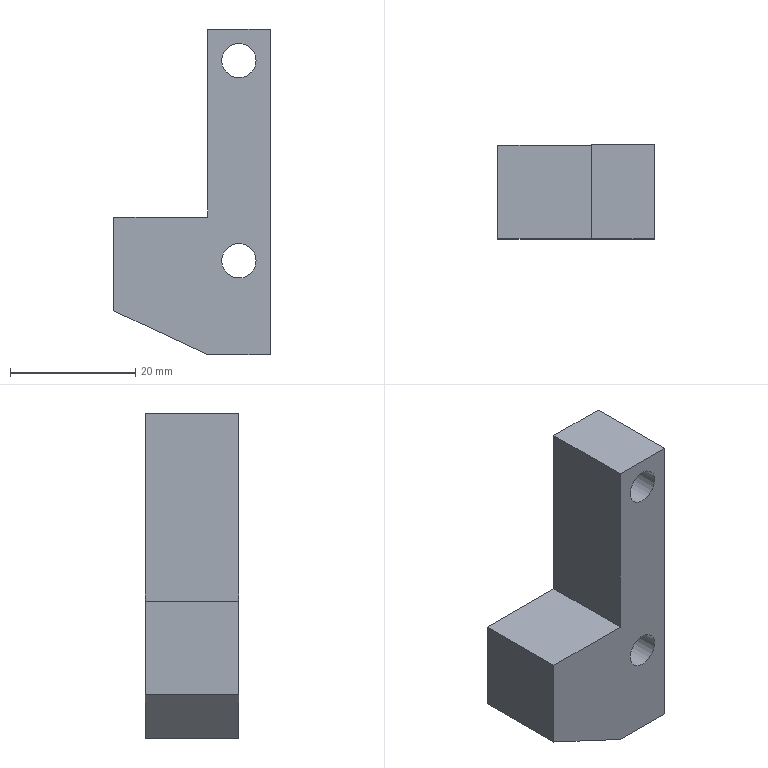Component | NX | NYLON_STOPPER_BLOCK_2 | 1 solid | 11 faces | box 25 x 15 x 52 mm | volume 11250 mm3 | plane 9 | cylinder 2 | commonest cylinder face diameters 5.5 x2
STEP:
#1=CARTESIAN_POINT('',(0.,0.,0.));
#2=DIRECTION('',(0.,0.,1.));
#3=DIRECTION('',(1.,0.,0.));
#4=AXIS2_PLACEMENT_3D('',#1,#2,#3);
#5=CARTESIAN_POINT('',(127.866,114.757,126.466));
#6=VERTEX_POINT('',#5);
#7=CARTESIAN_POINT('',(127.866,114.757,74.466));
#8=VERTEX_POINT('',#7);
#9=CARTESIAN_POINT('',(127.866,114.757,126.466));
#10=DIRECTION('',(0.,0.,-1.));
#11=VECTOR('',#10,1.);
#12=LINE('',#9,#11);
#13=CARTESIAN_POINT('',(127.866,129.757,126.466));
#14=DIRECTION('',(-1.,0.,0.));
#15=DIRECTION('',(0.,-1.,0.));
#16=AXIS2_PLACEMENT_3D('',#13,#14,#15);
#17=PLANE('',#16);
#18=CARTESIAN_POINT('',(15.,0.));
#19=DIRECTION('',(0.,-1.));
#20=VECTOR('',#19,1.);
#21=LINE('',#18,#20);
#22=(GEOMETRIC_REPRESENTATION_CONTEXT(2)PARAMETRIC_REPRESENTATION_CONTEXT()REPRESENTATION_CONTEXT('',''));
#23=DEFINITIONAL_REPRESENTATION('',(#21),#22);
#24=PCURVE('',#17,#23);
#25=CARTESIAN_POINT('',(122.866,114.757,89.466));
#26=DIRECTION('',(0.,1.,0.));
#27=DIRECTION('',(-1.,0.,0.));
#28=AXIS2_PLACEMENT_3D('',#25,#26,#27);
#29=PLANE('',#28);
#30=CARTESIAN_POINT('',(-5.,37.));
#31=DIRECTION('',(0.,-1.));
#32=VECTOR('',#31,1.);
#33=LINE('',#30,#32);
#34=(GEOMETRIC_REPRESENTATION_CONTEXT(2)PARAMETRIC_REPRESENTATION_CONTEXT()REPRESENTATION_CONTEXT('',''));
#35=DEFINITIONAL_REPRESENTATION('',(#33),#34);
#36=PCURVE('',#29,#35);
#37=SURFACE_CURVE('',#12,(#24,#36),.PCURVE_S1.);
#38=EDGE_CURVE('',#6,#8,#37,.T.);
#39=ORIENTED_EDGE('',*,*,#38,.T.);
#40=CARTESIAN_POINT('',(127.866,129.757,74.466));
#41=VERTEX_POINT('',#40);
#42=CARTESIAN_POINT('',(127.866,129.757,74.466));
#43=DIRECTION('',(0.,-1.,0.));
#44=VECTOR('',#43,1.);
#45=LINE('',#42,#44);
#46=CARTESIAN_POINT('',(0.,-52.));
#47=DIRECTION('',(1.,0.));
#48=VECTOR('',#47,1.);
#49=LINE('',#46,#48);
#50=(GEOMETRIC_REPRESENTATION_CONTEXT(2)PARAMETRIC_REPRESENTATION_CONTEXT()REPRESENTATION_CONTEXT('',''));
#51=DEFINITIONAL_REPRESENTATION('',(#49),#50);
#52=PCURVE('',#17,#51);
#53=CARTESIAN_POINT('',(127.866,129.757,74.466));
#54=DIRECTION('',(0.,0.,1.));
#55=DIRECTION('',(0.,1.,0.));
#56=AXIS2_PLACEMENT_3D('',#53,#54,#55);
#57=PLANE('',#56);
#58=CARTESIAN_POINT('',(0.,0.));
#59=DIRECTION('',(-1.,0.));
#60=VECTOR('',#59,1.);
#61=LINE('',#58,#60);
#62=(GEOMETRIC_REPRESENTATION_CONTEXT(2)PARAMETRIC_REPRESENTATION_CONTEXT()REPRESENTATION_CONTEXT('',''));
#63=DEFINITIONAL_REPRESENTATION('',(#61),#62);
#64=PCURVE('',#57,#63);
#65=SURFACE_CURVE('',#45,(#52,#64),.PCURVE_S1.);
#66=EDGE_CURVE('',#41,#8,#65,.T.);
#67=ORIENTED_EDGE('',*,*,#66,.F.);
#68=CARTESIAN_POINT('',(127.866,129.757,126.466));
#69=VERTEX_POINT('',#68);
#70=CARTESIAN_POINT('',(127.866,129.757,126.466));
#71=DIRECTION('',(0.,0.,-1.));
#72=VECTOR('',#71,1.);
#73=LINE('',#70,#72);
#74=CARTESIAN_POINT('',(0.,0.));
#75=DIRECTION('',(0.,-1.));
#76=VECTOR('',#75,1.);
#77=LINE('',#74,#76);
#78=(GEOMETRIC_REPRESENTATION_CONTEXT(2)PARAMETRIC_REPRESENTATION_CONTEXT()REPRESENTATION_CONTEXT('',''));
#79=DEFINITIONAL_REPRESENTATION('',(#77),#78);
#80=PCURVE('',#17,#79);
#81=CARTESIAN_POINT('',(122.866,129.757,89.466));
#82=DIRECTION('',(0.,1.,0.));
#83=DIRECTION('',(-1.,0.,0.));
#84=AXIS2_PLACEMENT_3D('',#81,#82,#83);
#85=PLANE('',#84);
#86=CARTESIAN_POINT('',(-5.,37.));
#87=DIRECTION('',(0.,-1.));
#88=VECTOR('',#87,1.);
#89=LINE('',#86,#88);
#90=(GEOMETRIC_REPRESENTATION_CONTEXT(2)PARAMETRIC_REPRESENTATION_CONTEXT()REPRESENTATION_CONTEXT('',''));
#91=DEFINITIONAL_REPRESENTATION('',(#89),#90);
#92=PCURVE('',#85,#91);
#93=SURFACE_CURVE('',#73,(#80,#92),.PCURVE_S1.);
#94=EDGE_CURVE('',#69,#41,#93,.T.);
#95=ORIENTED_EDGE('',*,*,#94,.F.);
#96=CARTESIAN_POINT('',(127.866,129.757,126.466));
#97=DIRECTION('',(0.,-1.,0.));
#98=VECTOR('',#97,1.);
#99=LINE('',#96,#98);
#100=CARTESIAN_POINT('',(0.,0.));
#101=DIRECTION('',(1.,0.));
#102=VECTOR('',#101,1.);
#103=LINE('',#100,#102);
#104=(GEOMETRIC_REPRESENTATION_CONTEXT(2)PARAMETRIC_REPRESENTATION_CONTEXT()REPRESENTATION_CONTEXT('',''));
#105=DEFINITIONAL_REPRESENTATION('',(#103),#104);
#106=PCURVE('',#17,#105);
#107=CARTESIAN_POINT('',(117.866,129.757,126.466));
#108=DIRECTION('',(0.,0.,-1.));
#109=DIRECTION('',(0.,-1.,0.));
#110=AXIS2_PLACEMENT_3D('',#107,#108,#109);
#111=PLANE('',#110);
#112=CARTESIAN_POINT('',(0.,-10.));
#113=DIRECTION('',(1.,0.));
#114=VECTOR('',#113,1.);
#115=LINE('',#112,#114);
#116=(GEOMETRIC_REPRESENTATION_CONTEXT(2)PARAMETRIC_REPRESENTATION_CONTEXT()REPRESENTATION_CONTEXT('',''));
#117=DEFINITIONAL_REPRESENTATION('',(#115),#116);
#118=PCURVE('',#111,#117);
#119=SURFACE_CURVE('',#99,(#106,#118),.PCURVE_S1.);
#120=EDGE_CURVE('',#69,#6,#119,.T.);
#121=ORIENTED_EDGE('',*,*,#120,.T.);
#122=EDGE_LOOP('',(#39,#67,#95,#121));
#123=FACE_BOUND('',#122,.T.);
#124=ADVANCED_FACE('',(#123),#17,.F.);
#125=CARTESIAN_POINT('',(117.866,114.757,74.466));
#126=VERTEX_POINT('',#125);
#127=CARTESIAN_POINT('',(127.866,114.757,74.466));
#128=DIRECTION('',(-1.,0.,0.));
#129=VECTOR('',#128,1.);
#130=LINE('',#127,#129);
#131=CARTESIAN_POINT('',(-15.,0.));
#132=DIRECTION('',(0.,1.));
#133=VECTOR('',#132,1.);
#134=LINE('',#131,#133);
#135=(GEOMETRIC_REPRESENTATION_CONTEXT(2)PARAMETRIC_REPRESENTATION_CONTEXT()REPRESENTATION_CONTEXT('',''));
#136=DEFINITIONAL_REPRESENTATION('',(#134),#135);
#137=PCURVE('',#57,#136);
#138=CARTESIAN_POINT('',(-5.,-15.));
#139=DIRECTION('',(1.,0.));
#140=VECTOR('',#139,1.);
#141=LINE('',#138,#140);
#142=(GEOMETRIC_REPRESENTATION_CONTEXT(2)PARAMETRIC_REPRESENTATION_CONTEXT()REPRESENTATION_CONTEXT('',''));
#143=DEFINITIONAL_REPRESENTATION('',(#141),#142);
#144=PCURVE('',#29,#143);
#145=SURFACE_CURVE('',#130,(#137,#144),.PCURVE_S1.);
#146=EDGE_CURVE('',#8,#126,#145,.T.);
#147=ORIENTED_EDGE('',*,*,#146,.T.);
#148=CARTESIAN_POINT('',(117.866,129.757,74.466));
#149=VERTEX_POINT('',#148);
#150=CARTESIAN_POINT('',(117.866,129.757,74.466));
#151=DIRECTION('',(0.,-1.,0.));
#152=VECTOR('',#151,1.);
#153=LINE('',#150,#152);
#154=CARTESIAN_POINT('',(0.,10.));
#155=DIRECTION('',(-1.,0.));
#156=VECTOR('',#155,1.);
#157=LINE('',#154,#156);
#158=(GEOMETRIC_REPRESENTATION_CONTEXT(2)PARAMETRIC_REPRESENTATION_CONTEXT()REPRESENTATION_CONTEXT('',''));
#159=DEFINITIONAL_REPRESENTATION('',(#157),#158);
#160=PCURVE('',#57,#159);
#161=CARTESIAN_POINT('',(117.866,129.757,74.466));
#162=DIRECTION('',(0.4229,0.,0.9062));
#163=DIRECTION('',(0.9062,0.,-0.4229));
#164=AXIS2_PLACEMENT_3D('',#161,#162,#163);
#165=PLANE('',#164);
#166=CARTESIAN_POINT('',(0.,0.));
#167=DIRECTION('',(0.,-1.));
#168=VECTOR('',#167,1.);
#169=LINE('',#166,#168);
#170=(GEOMETRIC_REPRESENTATION_CONTEXT(2)PARAMETRIC_REPRESENTATION_CONTEXT()REPRESENTATION_CONTEXT('',''));
#171=DEFINITIONAL_REPRESENTATION('',(#169),#170);
#172=PCURVE('',#165,#171);
#173=SURFACE_CURVE('',#153,(#160,#172),.PCURVE_S1.);
#174=EDGE_CURVE('',#149,#126,#173,.T.);
#175=ORIENTED_EDGE('',*,*,#174,.F.);
#176=CARTESIAN_POINT('',(127.866,129.757,74.466));
#177=DIRECTION('',(-1.,0.,0.));
#178=VECTOR('',#177,1.);
#179=LINE('',#176,#178);
#180=CARTESIAN_POINT('',(0.,0.));
#181=DIRECTION('',(0.,1.));
#182=VECTOR('',#181,1.);
#183=LINE('',#180,#182);
#184=(GEOMETRIC_REPRESENTATION_CONTEXT(2)PARAMETRIC_REPRESENTATION_CONTEXT()REPRESENTATION_CONTEXT('',''));
#185=DEFINITIONAL_REPRESENTATION('',(#183),#184);
#186=PCURVE('',#57,#185);
#187=CARTESIAN_POINT('',(-5.,-15.));
#188=DIRECTION('',(1.,0.));
#189=VECTOR('',#188,1.);
#190=LINE('',#187,#189);
#191=(GEOMETRIC_REPRESENTATION_CONTEXT(2)PARAMETRIC_REPRESENTATION_CONTEXT()REPRESENTATION_CONTEXT('',''));
#192=DEFINITIONAL_REPRESENTATION('',(#190),#191);
#193=PCURVE('',#85,#192);
#194=SURFACE_CURVE('',#179,(#186,#193),.PCURVE_S1.);
#195=EDGE_CURVE('',#41,#149,#194,.T.);
#196=ORIENTED_EDGE('',*,*,#195,.F.);
#197=ORIENTED_EDGE('',*,*,#66,.T.);
#198=EDGE_LOOP('',(#147,#175,#196,#197));
#199=FACE_BOUND('',#198,.T.);
#200=ADVANCED_FACE('',(#199),#57,.F.);
#201=CARTESIAN_POINT('',(102.866,114.757,81.466));
#202=VERTEX_POINT('',#201);
#203=CARTESIAN_POINT('',(117.866,114.757,74.466));
#204=DIRECTION('',(-0.9062,0.,0.4229));
#205=VECTOR('',#204,1.);
#206=LINE('',#203,#205);
#207=CARTESIAN_POINT('',(0.,-15.));
#208=DIRECTION('',(-1.,0.));
#209=VECTOR('',#208,1.);
#210=LINE('',#207,#209);
#211=(GEOMETRIC_REPRESENTATION_CONTEXT(2)PARAMETRIC_REPRESENTATION_CONTEXT()REPRESENTATION_CONTEXT('',''));
#212=DEFINITIONAL_REPRESENTATION('',(#210),#211);
#213=PCURVE('',#165,#212);
#214=CARTESIAN_POINT('',(5.,-15.));
#215=DIRECTION('',(0.9062,0.4229));
#216=VECTOR('',#215,1.);
#217=LINE('',#214,#216);
#218=(GEOMETRIC_REPRESENTATION_CONTEXT(2)PARAMETRIC_REPRESENTATION_CONTEXT()REPRESENTATION_CONTEXT('',''));
#219=DEFINITIONAL_REPRESENTATION('',(#217),#218);
#220=PCURVE('',#29,#219);
#221=SURFACE_CURVE('',#206,(#213,#220),.PCURVE_S1.);
#222=EDGE_CURVE('',#126,#202,#221,.T.);
#223=ORIENTED_EDGE('',*,*,#222,.T.);
#224=CARTESIAN_POINT('',(102.866,129.757,81.466));
#225=VERTEX_POINT('',#224);
#226=CARTESIAN_POINT('',(102.866,129.757,81.466));
#227=DIRECTION('',(0.,-1.,0.));
#228=VECTOR('',#227,1.);
#229=LINE('',#226,#228);
#230=CARTESIAN_POINT('',(-16.553,0.));
#231=DIRECTION('',(0.,-1.));
#232=VECTOR('',#231,1.);
#233=LINE('',#230,#232);
#234=(GEOMETRIC_REPRESENTATION_CONTEXT(2)PARAMETRIC_REPRESENTATION_CONTEXT()REPRESENTATION_CONTEXT('',''));
#235=DEFINITIONAL_REPRESENTATION('',(#233),#234);
#236=PCURVE('',#165,#235);
#237=CARTESIAN_POINT('',(102.866,129.757,81.466));
#238=DIRECTION('',(1.,0.,-0.));
#239=DIRECTION('',(-0.,0.,-1.));
#240=AXIS2_PLACEMENT_3D('',#237,#238,#239);
#241=PLANE('',#240);
#242=CARTESIAN_POINT('',(0.,0.));
#243=DIRECTION('',(0.,-1.));
#244=VECTOR('',#243,1.);
#245=LINE('',#242,#244);
#246=(GEOMETRIC_REPRESENTATION_CONTEXT(2)PARAMETRIC_REPRESENTATION_CONTEXT()REPRESENTATION_CONTEXT('',''));
#247=DEFINITIONAL_REPRESENTATION('',(#245),#246);
#248=PCURVE('',#241,#247);
#249=SURFACE_CURVE('',#229,(#236,#248),.PCURVE_S1.);
#250=EDGE_CURVE('',#225,#202,#249,.T.);
#251=ORIENTED_EDGE('',*,*,#250,.F.);
#252=CARTESIAN_POINT('',(117.866,129.757,74.466));
#253=DIRECTION('',(-0.9062,0.,0.4229));
#254=VECTOR('',#253,1.);
#255=LINE('',#252,#254);
#256=CARTESIAN_POINT('',(0.,0.));
#257=DIRECTION('',(-1.,0.));
#258=VECTOR('',#257,1.);
#259=LINE('',#256,#258);
#260=(GEOMETRIC_REPRESENTATION_CONTEXT(2)PARAMETRIC_REPRESENTATION_CONTEXT()REPRESENTATION_CONTEXT('',''));
#261=DEFINITIONAL_REPRESENTATION('',(#259),#260);
#262=PCURVE('',#165,#261);
#263=CARTESIAN_POINT('',(5.,-15.));
#264=DIRECTION('',(0.9062,0.4229));
#265=VECTOR('',#264,1.);
#266=LINE('',#263,#265);
#267=(GEOMETRIC_REPRESENTATION_CONTEXT(2)PARAMETRIC_REPRESENTATION_CONTEXT()REPRESENTATION_CONTEXT('',''));
#268=DEFINITIONAL_REPRESENTATION('',(#266),#267);
#269=PCURVE('',#85,#268);
#270=SURFACE_CURVE('',#255,(#262,#269),.PCURVE_S1.);
#271=EDGE_CURVE('',#149,#225,#270,.T.);
#272=ORIENTED_EDGE('',*,*,#271,.F.);
#273=ORIENTED_EDGE('',*,*,#174,.T.);
#274=EDGE_LOOP('',(#223,#251,#272,#273));
#275=FACE_BOUND('',#274,.T.);
#276=ADVANCED_FACE('',(#275),#165,.F.);
#277=CARTESIAN_POINT('',(102.866,114.757,96.466));
#278=VERTEX_POINT('',#277);
#279=CARTESIAN_POINT('',(102.866,114.757,81.466));
#280=DIRECTION('',(0.,0.,1.));
#281=VECTOR('',#280,1.);
#282=LINE('',#279,#281);
#283=CARTESIAN_POINT('',(0.,-15.));
#284=DIRECTION('',(-1.,0.));
#285=VECTOR('',#284,1.);
#286=LINE('',#283,#285);
#287=(GEOMETRIC_REPRESENTATION_CONTEXT(2)PARAMETRIC_REPRESENTATION_CONTEXT()REPRESENTATION_CONTEXT('',''));
#288=DEFINITIONAL_REPRESENTATION('',(#286),#287);
#289=PCURVE('',#241,#288);
#290=CARTESIAN_POINT('',(20.,-8.));
#291=DIRECTION('',(-0.,1.));
#292=VECTOR('',#291,1.);
#293=LINE('',#290,#292);
#294=(GEOMETRIC_REPRESENTATION_CONTEXT(2)PARAMETRIC_REPRESENTATION_CONTEXT()REPRESENTATION_CONTEXT('',''));
#295=DEFINITIONAL_REPRESENTATION('',(#293),#294);
#296=PCURVE('',#29,#295);
#297=SURFACE_CURVE('',#282,(#289,#296),.PCURVE_S1.);
#298=EDGE_CURVE('',#202,#278,#297,.T.);
#299=ORIENTED_EDGE('',*,*,#298,.T.);
#300=CARTESIAN_POINT('',(102.866,129.757,96.466));
#301=VERTEX_POINT('',#300);
#302=CARTESIAN_POINT('',(102.866,129.757,96.466));
#303=DIRECTION('',(0.,-1.,0.));
#304=VECTOR('',#303,1.);
#305=LINE('',#302,#304);
#306=CARTESIAN_POINT('',(-15.,0.));
#307=DIRECTION('',(0.,-1.));
#308=VECTOR('',#307,1.);
#309=LINE('',#306,#308);
#310=(GEOMETRIC_REPRESENTATION_CONTEXT(2)PARAMETRIC_REPRESENTATION_CONTEXT()REPRESENTATION_CONTEXT('',''));
#311=DEFINITIONAL_REPRESENTATION('',(#309),#310);
#312=PCURVE('',#241,#311);
#313=CARTESIAN_POINT('',(102.866,129.757,96.466));
#314=DIRECTION('',(0.,0.,-1.));
#315=DIRECTION('',(0.,-1.,0.));
#316=AXIS2_PLACEMENT_3D('',#313,#314,#315);
#317=PLANE('',#316);
#318=CARTESIAN_POINT('',(0.,0.));
#319=DIRECTION('',(1.,0.));
#320=VECTOR('',#319,1.);
#321=LINE('',#318,#320);
#322=(GEOMETRIC_REPRESENTATION_CONTEXT(2)PARAMETRIC_REPRESENTATION_CONTEXT()REPRESENTATION_CONTEXT('',''));
#323=DEFINITIONAL_REPRESENTATION('',(#321),#322);
#324=PCURVE('',#317,#323);
#325=SURFACE_CURVE('',#305,(#312,#324),.PCURVE_S1.);
#326=EDGE_CURVE('',#301,#278,#325,.T.);
#327=ORIENTED_EDGE('',*,*,#326,.F.);
#328=CARTESIAN_POINT('',(102.866,129.757,81.466));
#329=DIRECTION('',(0.,0.,1.));
#330=VECTOR('',#329,1.);
#331=LINE('',#328,#330);
#332=CARTESIAN_POINT('',(0.,0.));
#333=DIRECTION('',(-1.,0.));
#334=VECTOR('',#333,1.);
#335=LINE('',#332,#334);
#336=(GEOMETRIC_REPRESENTATION_CONTEXT(2)PARAMETRIC_REPRESENTATION_CONTEXT()REPRESENTATION_CONTEXT('',''));
#337=DEFINITIONAL_REPRESENTATION('',(#335),#336);
#338=PCURVE('',#241,#337);
#339=CARTESIAN_POINT('',(20.,-8.));
#340=DIRECTION('',(-0.,1.));
#341=VECTOR('',#340,1.);
#342=LINE('',#339,#341);
#343=(GEOMETRIC_REPRESENTATION_CONTEXT(2)PARAMETRIC_REPRESENTATION_CONTEXT()REPRESENTATION_CONTEXT('',''));
#344=DEFINITIONAL_REPRESENTATION('',(#342),#343);
#345=PCURVE('',#85,#344);
#346=SURFACE_CURVE('',#331,(#338,#345),.PCURVE_S1.);
#347=EDGE_CURVE('',#225,#301,#346,.T.);
#348=ORIENTED_EDGE('',*,*,#347,.F.);
#349=ORIENTED_EDGE('',*,*,#250,.T.);
#350=EDGE_LOOP('',(#299,#327,#348,#349));
#351=FACE_BOUND('',#350,.T.);
#352=ADVANCED_FACE('',(#351),#241,.F.);
#353=CARTESIAN_POINT('',(117.866,114.757,96.466));
#354=VERTEX_POINT('',#353);
#355=CARTESIAN_POINT('',(102.866,114.757,96.466));
#356=DIRECTION('',(1.,0.,0.));
#357=VECTOR('',#356,1.);
#358=LINE('',#355,#357);
#359=CARTESIAN_POINT('',(15.,0.));
#360=DIRECTION('',(0.,-1.));
#361=VECTOR('',#360,1.);
#362=LINE('',#359,#361);
#363=(GEOMETRIC_REPRESENTATION_CONTEXT(2)PARAMETRIC_REPRESENTATION_CONTEXT()REPRESENTATION_CONTEXT('',''));
#364=DEFINITIONAL_REPRESENTATION('',(#362),#363);
#365=PCURVE('',#317,#364);
#366=CARTESIAN_POINT('',(20.,7.));
#367=DIRECTION('',(-1.,0.));
#368=VECTOR('',#367,1.);
#369=LINE('',#366,#368);
#370=(GEOMETRIC_REPRESENTATION_CONTEXT(2)PARAMETRIC_REPRESENTATION_CONTEXT()REPRESENTATION_CONTEXT('',''));
#371=DEFINITIONAL_REPRESENTATION('',(#369),#370);
#372=PCURVE('',#29,#371);
#373=SURFACE_CURVE('',#358,(#365,#372),.PCURVE_S1.);
#374=EDGE_CURVE('',#278,#354,#373,.T.);
#375=ORIENTED_EDGE('',*,*,#374,.T.);
#376=CARTESIAN_POINT('',(117.866,129.757,96.466));
#377=VERTEX_POINT('',#376);
#378=CARTESIAN_POINT('',(117.866,129.757,96.466));
#379=DIRECTION('',(0.,-1.,0.));
#380=VECTOR('',#379,1.);
#381=LINE('',#378,#380);
#382=CARTESIAN_POINT('',(0.,-15.));
#383=DIRECTION('',(1.,0.));
#384=VECTOR('',#383,1.);
#385=LINE('',#382,#384);
#386=(GEOMETRIC_REPRESENTATION_CONTEXT(2)PARAMETRIC_REPRESENTATION_CONTEXT()REPRESENTATION_CONTEXT('',''));
#387=DEFINITIONAL_REPRESENTATION('',(#385),#386);
#388=PCURVE('',#317,#387);
#389=CARTESIAN_POINT('',(117.866,129.757,96.466));
#390=DIRECTION('',(1.,0.,-0.));
#391=DIRECTION('',(-0.,0.,-1.));
#392=AXIS2_PLACEMENT_3D('',#389,#390,#391);
#393=PLANE('',#392);
#394=CARTESIAN_POINT('',(0.,0.));
#395=DIRECTION('',(0.,-1.));
#396=VECTOR('',#395,1.);
#397=LINE('',#394,#396);
#398=(GEOMETRIC_REPRESENTATION_CONTEXT(2)PARAMETRIC_REPRESENTATION_CONTEXT()REPRESENTATION_CONTEXT('',''));
#399=DEFINITIONAL_REPRESENTATION('',(#397),#398);
#400=PCURVE('',#393,#399);
#401=SURFACE_CURVE('',#381,(#388,#400),.PCURVE_S1.);
#402=EDGE_CURVE('',#377,#354,#401,.T.);
#403=ORIENTED_EDGE('',*,*,#402,.F.);
#404=CARTESIAN_POINT('',(102.866,129.757,96.466));
#405=DIRECTION('',(1.,0.,0.));
#406=VECTOR('',#405,1.);
#407=LINE('',#404,#406);
#408=CARTESIAN_POINT('',(0.,0.));
#409=DIRECTION('',(0.,-1.));
#410=VECTOR('',#409,1.);
#411=LINE('',#408,#410);
#412=(GEOMETRIC_REPRESENTATION_CONTEXT(2)PARAMETRIC_REPRESENTATION_CONTEXT()REPRESENTATION_CONTEXT('',''));
#413=DEFINITIONAL_REPRESENTATION('',(#411),#412);
#414=PCURVE('',#317,#413);
#415=CARTESIAN_POINT('',(20.,7.));
#416=DIRECTION('',(-1.,0.));
#417=VECTOR('',#416,1.);
#418=LINE('',#415,#417);
#419=(GEOMETRIC_REPRESENTATION_CONTEXT(2)PARAMETRIC_REPRESENTATION_CONTEXT()REPRESENTATION_CONTEXT('',''));
#420=DEFINITIONAL_REPRESENTATION('',(#418),#419);
#421=PCURVE('',#85,#420);
#422=SURFACE_CURVE('',#407,(#414,#421),.PCURVE_S1.);
#423=EDGE_CURVE('',#301,#377,#422,.T.);
#424=ORIENTED_EDGE('',*,*,#423,.F.);
#425=ORIENTED_EDGE('',*,*,#326,.T.);
#426=EDGE_LOOP('',(#375,#403,#424,#425));
#427=FACE_BOUND('',#426,.T.);
#428=ADVANCED_FACE('',(#427),#317,.F.);
#429=CARTESIAN_POINT('',(117.866,114.757,126.466));
#430=VERTEX_POINT('',#429);
#431=CARTESIAN_POINT('',(117.866,114.757,96.466));
#432=DIRECTION('',(0.,0.,1.));
#433=VECTOR('',#432,1.);
#434=LINE('',#431,#433);
#435=CARTESIAN_POINT('',(0.,-15.));
#436=DIRECTION('',(-1.,0.));
#437=VECTOR('',#436,1.);
#438=LINE('',#435,#437);
#439=(GEOMETRIC_REPRESENTATION_CONTEXT(2)PARAMETRIC_REPRESENTATION_CONTEXT()REPRESENTATION_CONTEXT('',''));
#440=DEFINITIONAL_REPRESENTATION('',(#438),#439);
#441=PCURVE('',#393,#440);
#442=CARTESIAN_POINT('',(5.,7.));
#443=DIRECTION('',(-0.,1.));
#444=VECTOR('',#443,1.);
#445=LINE('',#442,#444);
#446=(GEOMETRIC_REPRESENTATION_CONTEXT(2)PARAMETRIC_REPRESENTATION_CONTEXT()REPRESENTATION_CONTEXT('',''));
#447=DEFINITIONAL_REPRESENTATION('',(#445),#446);
#448=PCURVE('',#29,#447);
#449=SURFACE_CURVE('',#434,(#441,#448),.PCURVE_S1.);
#450=EDGE_CURVE('',#354,#430,#449,.T.);
#451=ORIENTED_EDGE('',*,*,#450,.T.);
#452=CARTESIAN_POINT('',(117.866,129.757,126.466));
#453=VERTEX_POINT('',#452);
#454=CARTESIAN_POINT('',(117.866,129.757,126.466));
#455=DIRECTION('',(0.,-1.,0.));
#456=VECTOR('',#455,1.);
#457=LINE('',#454,#456);
#458=CARTESIAN_POINT('',(-30.,0.));
#459=DIRECTION('',(0.,-1.));
#460=VECTOR('',#459,1.);
#461=LINE('',#458,#460);
#462=(GEOMETRIC_REPRESENTATION_CONTEXT(2)PARAMETRIC_REPRESENTATION_CONTEXT()REPRESENTATION_CONTEXT('',''));
#463=DEFINITIONAL_REPRESENTATION('',(#461),#462);
#464=PCURVE('',#393,#463);
#465=CARTESIAN_POINT('',(0.,0.));
#466=DIRECTION('',(1.,0.));
#467=VECTOR('',#466,1.);
#468=LINE('',#465,#467);
#469=(GEOMETRIC_REPRESENTATION_CONTEXT(2)PARAMETRIC_REPRESENTATION_CONTEXT()REPRESENTATION_CONTEXT('',''));
#470=DEFINITIONAL_REPRESENTATION('',(#468),#469);
#471=PCURVE('',#111,#470);
#472=SURFACE_CURVE('',#457,(#464,#471),.PCURVE_S1.);
#473=EDGE_CURVE('',#453,#430,#472,.T.);
#474=ORIENTED_EDGE('',*,*,#473,.F.);
#475=CARTESIAN_POINT('',(117.866,129.757,96.466));
#476=DIRECTION('',(0.,0.,1.));
#477=VECTOR('',#476,1.);
#478=LINE('',#475,#477);
#479=CARTESIAN_POINT('',(0.,0.));
#480=DIRECTION('',(-1.,0.));
#481=VECTOR('',#480,1.);
#482=LINE('',#479,#481);
#483=(GEOMETRIC_REPRESENTATION_CONTEXT(2)PARAMETRIC_REPRESENTATION_CONTEXT()REPRESENTATION_CONTEXT('',''));
#484=DEFINITIONAL_REPRESENTATION('',(#482),#483);
#485=PCURVE('',#393,#484);
#486=CARTESIAN_POINT('',(5.,7.));
#487=DIRECTION('',(-0.,1.));
#488=VECTOR('',#487,1.);
#489=LINE('',#486,#488);
#490=(GEOMETRIC_REPRESENTATION_CONTEXT(2)PARAMETRIC_REPRESENTATION_CONTEXT()REPRESENTATION_CONTEXT('',''));
#491=DEFINITIONAL_REPRESENTATION('',(#489),#490);
#492=PCURVE('',#85,#491);
#493=SURFACE_CURVE('',#478,(#485,#492),.PCURVE_S1.);
#494=EDGE_CURVE('',#377,#453,#493,.T.);
#495=ORIENTED_EDGE('',*,*,#494,.F.);
#496=ORIENTED_EDGE('',*,*,#402,.T.);
#497=EDGE_LOOP('',(#451,#474,#495,#496));
#498=FACE_BOUND('',#497,.T.);
#499=ADVANCED_FACE('',(#498),#393,.F.);
#500=CARTESIAN_POINT('',(120.116,129.757,89.466));
#501=VERTEX_POINT('',#500);
#502=CARTESIAN_POINT('',(122.866,129.757,89.466));
#503=DIRECTION('',(0.,1.,0.));
#504=DIRECTION('',(-1.,0.,0.));
#505=AXIS2_PLACEMENT_3D('',#502,#503,#504);
#506=CIRCLE('',#505,2.75);
#507=CARTESIAN_POINT('',(122.866,129.757,89.466));
#508=DIRECTION('',(0.,-1.,0.));
#509=DIRECTION('',(1.,0.,0.));
#510=AXIS2_PLACEMENT_3D('',#507,#508,#509);
#511=CYLINDRICAL_SURFACE('',#510,2.75);
#512=CARTESIAN_POINT('',(9.425,0.));
#513=DIRECTION('',(-1.,0.));
#514=VECTOR('',#513,1.);
#515=LINE('',#512,#514);
#516=(GEOMETRIC_REPRESENTATION_CONTEXT(2)PARAMETRIC_REPRESENTATION_CONTEXT()REPRESENTATION_CONTEXT('',''));
#517=DEFINITIONAL_REPRESENTATION('',(#515),#516);
#518=PCURVE('',#511,#517);
#519=CARTESIAN_POINT('',(0.,0.));
#520=DIRECTION('',(1.,0.));
#521=AXIS2_PLACEMENT_2D('',#519,#520);
#522=CIRCLE('',#521,2.75);
#523=(GEOMETRIC_REPRESENTATION_CONTEXT(2)PARAMETRIC_REPRESENTATION_CONTEXT()REPRESENTATION_CONTEXT('',''));
#524=DEFINITIONAL_REPRESENTATION('',(#522),#523);
#525=PCURVE('',#85,#524);
#526=SURFACE_CURVE('',#506,(#518,#525),.PCURVE_S1.);
#527=EDGE_CURVE('',#501,#501,#526,.T.);
#528=ORIENTED_EDGE('',*,*,#527,.F.);
#529=CARTESIAN_POINT('',(120.116,114.757,89.466));
#530=VERTEX_POINT('',#529);
#531=CARTESIAN_POINT('',(120.116,129.757,89.466));
#532=CARTESIAN_POINT('',(120.116,114.757,89.466));
#533=B_SPLINE_CURVE_WITH_KNOTS('',1,(#531,#532),.UNSPECIFIED.,.F.,.F.,(2,2),(0.,15.),.PIECEWISE_BEZIER_KNOTS.);
#534=CARTESIAN_POINT('',(9.425,0.));
#535=DIRECTION('',(0.,1.));
#536=VECTOR('',#535,1.);
#537=LINE('',#534,#536);
#538=(GEOMETRIC_REPRESENTATION_CONTEXT(2)PARAMETRIC_REPRESENTATION_CONTEXT()REPRESENTATION_CONTEXT('',''));
#539=DEFINITIONAL_REPRESENTATION('',(#537),#538);
#540=PCURVE('',#511,#539);
#541=CARTESIAN_POINT('',(3.142,0.));
#542=DIRECTION('',(0.,1.));
#543=VECTOR('',#542,1.);
#544=LINE('',#541,#543);
#545=(GEOMETRIC_REPRESENTATION_CONTEXT(2)PARAMETRIC_REPRESENTATION_CONTEXT()REPRESENTATION_CONTEXT('',''));
#546=DEFINITIONAL_REPRESENTATION('',(#544),#545);
#547=PCURVE('',#511,#546);
#548=SEAM_CURVE('',#533,(#540,#547),.PCURVE_S1.);
#549=EDGE_CURVE('',#501,#530,#548,.T.);
#550=ORIENTED_EDGE('',*,*,#549,.T.);
#551=CARTESIAN_POINT('',(122.866,114.757,89.466));
#552=DIRECTION('',(0.,1.,0.));
#553=DIRECTION('',(-1.,0.,0.));
#554=AXIS2_PLACEMENT_3D('',#551,#552,#553);
#555=CIRCLE('',#554,2.75);
#556=CARTESIAN_POINT('',(9.425,15.));
#557=DIRECTION('',(-1.,0.));
#558=VECTOR('',#557,1.);
#559=LINE('',#556,#558);
#560=(GEOMETRIC_REPRESENTATION_CONTEXT(2)PARAMETRIC_REPRESENTATION_CONTEXT()REPRESENTATION_CONTEXT('',''));
#561=DEFINITIONAL_REPRESENTATION('',(#559),#560);
#562=PCURVE('',#511,#561);
#563=CARTESIAN_POINT('',(0.,0.));
#564=DIRECTION('',(1.,0.));
#565=AXIS2_PLACEMENT_2D('',#563,#564);
#566=CIRCLE('',#565,2.75);
#567=(GEOMETRIC_REPRESENTATION_CONTEXT(2)PARAMETRIC_REPRESENTATION_CONTEXT()REPRESENTATION_CONTEXT('',''));
#568=DEFINITIONAL_REPRESENTATION('',(#566),#567);
#569=PCURVE('',#29,#568);
#570=SURFACE_CURVE('',#555,(#562,#569),.PCURVE_S1.);
#571=EDGE_CURVE('',#530,#530,#570,.T.);
#572=ORIENTED_EDGE('',*,*,#571,.T.);
#573=ORIENTED_EDGE('',*,*,#549,.F.);
#574=EDGE_LOOP('',(#528,#550,#572,#573));
#575=FACE_BOUND('',#574,.F.);
#576=ADVANCED_FACE('',(#575),#511,.F.);
#577=CARTESIAN_POINT('',(117.866,114.757,126.466));
#578=DIRECTION('',(1.,0.,0.));
#579=VECTOR('',#578,1.);
#580=LINE('',#577,#579);
#581=CARTESIAN_POINT('',(15.,0.));
#582=DIRECTION('',(0.,-1.));
#583=VECTOR('',#582,1.);
#584=LINE('',#581,#583);
#585=(GEOMETRIC_REPRESENTATION_CONTEXT(2)PARAMETRIC_REPRESENTATION_CONTEXT()REPRESENTATION_CONTEXT('',''));
#586=DEFINITIONAL_REPRESENTATION('',(#584),#585);
#587=PCURVE('',#111,#586);
#588=CARTESIAN_POINT('',(5.,37.));
#589=DIRECTION('',(-1.,0.));
#590=VECTOR('',#589,1.);
#591=LINE('',#588,#590);
#592=(GEOMETRIC_REPRESENTATION_CONTEXT(2)PARAMETRIC_REPRESENTATION_CONTEXT()REPRESENTATION_CONTEXT('',''));
#593=DEFINITIONAL_REPRESENTATION('',(#591),#592);
#594=PCURVE('',#29,#593);
#595=SURFACE_CURVE('',#580,(#587,#594),.PCURVE_S1.);
#596=EDGE_CURVE('',#430,#6,#595,.T.);
#597=ORIENTED_EDGE('',*,*,#596,.T.);
#598=ORIENTED_EDGE('',*,*,#120,.F.);
#599=CARTESIAN_POINT('',(117.866,129.757,126.466));
#600=DIRECTION('',(1.,0.,0.));
#601=VECTOR('',#600,1.);
#602=LINE('',#599,#601);
#603=CARTESIAN_POINT('',(0.,0.));
#604=DIRECTION('',(0.,-1.));
#605=VECTOR('',#604,1.);
#606=LINE('',#603,#605);
#607=(GEOMETRIC_REPRESENTATION_CONTEXT(2)PARAMETRIC_REPRESENTATION_CONTEXT()REPRESENTATION_CONTEXT('',''));
#608=DEFINITIONAL_REPRESENTATION('',(#606),#607);
#609=PCURVE('',#111,#608);
#610=CARTESIAN_POINT('',(5.,37.));
#611=DIRECTION('',(-1.,0.));
#612=VECTOR('',#611,1.);
#613=LINE('',#610,#612);
#614=(GEOMETRIC_REPRESENTATION_CONTEXT(2)PARAMETRIC_REPRESENTATION_CONTEXT()REPRESENTATION_CONTEXT('',''));
#615=DEFINITIONAL_REPRESENTATION('',(#613),#614);
#616=PCURVE('',#85,#615);
#617=SURFACE_CURVE('',#602,(#609,#616),.PCURVE_S1.);
#618=EDGE_CURVE('',#453,#69,#617,.T.);
#619=ORIENTED_EDGE('',*,*,#618,.F.);
#620=ORIENTED_EDGE('',*,*,#473,.T.);
#621=EDGE_LOOP('',(#597,#598,#619,#620));
#622=FACE_BOUND('',#621,.T.);
#623=ADVANCED_FACE('',(#622),#111,.F.);
#624=CARTESIAN_POINT('',(120.116,129.757,121.466));
#625=VERTEX_POINT('',#624);
#626=CARTESIAN_POINT('',(122.866,129.757,121.466));
#627=DIRECTION('',(0.,1.,0.));
#628=DIRECTION('',(-1.,0.,0.));
#629=AXIS2_PLACEMENT_3D('',#626,#627,#628);
#630=CIRCLE('',#629,2.75);
#631=CARTESIAN_POINT('',(122.866,129.757,121.466));
#632=DIRECTION('',(0.,-1.,0.));
#633=DIRECTION('',(1.,0.,0.));
#634=AXIS2_PLACEMENT_3D('',#631,#632,#633);
#635=CYLINDRICAL_SURFACE('',#634,2.75);
#636=CARTESIAN_POINT('',(9.425,0.));
#637=DIRECTION('',(-1.,0.));
#638=VECTOR('',#637,1.);
#639=LINE('',#636,#638);
#640=(GEOMETRIC_REPRESENTATION_CONTEXT(2)PARAMETRIC_REPRESENTATION_CONTEXT()REPRESENTATION_CONTEXT('',''));
#641=DEFINITIONAL_REPRESENTATION('',(#639),#640);
#642=PCURVE('',#635,#641);
#643=CARTESIAN_POINT('',(0.,32.));
#644=DIRECTION('',(1.,0.));
#645=AXIS2_PLACEMENT_2D('',#643,#644);
#646=CIRCLE('',#645,2.75);
#647=(GEOMETRIC_REPRESENTATION_CONTEXT(2)PARAMETRIC_REPRESENTATION_CONTEXT()REPRESENTATION_CONTEXT('',''));
#648=DEFINITIONAL_REPRESENTATION('',(#646),#647);
#649=PCURVE('',#85,#648);
#650=SURFACE_CURVE('',#630,(#642,#649),.PCURVE_S1.);
#651=EDGE_CURVE('',#625,#625,#650,.T.);
#652=ORIENTED_EDGE('',*,*,#651,.F.);
#653=CARTESIAN_POINT('',(120.116,114.757,121.466));
#654=VERTEX_POINT('',#653);
#655=CARTESIAN_POINT('',(120.116,129.757,121.466));
#656=CARTESIAN_POINT('',(120.116,114.757,121.466));
#657=B_SPLINE_CURVE_WITH_KNOTS('',1,(#655,#656),.UNSPECIFIED.,.F.,.F.,(2,2),(0.,15.),.PIECEWISE_BEZIER_KNOTS.);
#658=CARTESIAN_POINT('',(9.425,0.));
#659=DIRECTION('',(0.,1.));
#660=VECTOR('',#659,1.);
#661=LINE('',#658,#660);
#662=(GEOMETRIC_REPRESENTATION_CONTEXT(2)PARAMETRIC_REPRESENTATION_CONTEXT()REPRESENTATION_CONTEXT('',''));
#663=DEFINITIONAL_REPRESENTATION('',(#661),#662);
#664=PCURVE('',#635,#663);
#665=CARTESIAN_POINT('',(3.142,0.));
#666=DIRECTION('',(0.,1.));
#667=VECTOR('',#666,1.);
#668=LINE('',#665,#667);
#669=(GEOMETRIC_REPRESENTATION_CONTEXT(2)PARAMETRIC_REPRESENTATION_CONTEXT()REPRESENTATION_CONTEXT('',''));
#670=DEFINITIONAL_REPRESENTATION('',(#668),#669);
#671=PCURVE('',#635,#670);
#672=SEAM_CURVE('',#657,(#664,#671),.PCURVE_S1.);
#673=EDGE_CURVE('',#625,#654,#672,.T.);
#674=ORIENTED_EDGE('',*,*,#673,.T.);
#675=CARTESIAN_POINT('',(122.866,114.757,121.466));
#676=DIRECTION('',(0.,1.,0.));
#677=DIRECTION('',(-1.,0.,0.));
#678=AXIS2_PLACEMENT_3D('',#675,#676,#677);
#679=CIRCLE('',#678,2.75);
#680=CARTESIAN_POINT('',(9.425,15.));
#681=DIRECTION('',(-1.,0.));
#682=VECTOR('',#681,1.);
#683=LINE('',#680,#682);
#684=(GEOMETRIC_REPRESENTATION_CONTEXT(2)PARAMETRIC_REPRESENTATION_CONTEXT()REPRESENTATION_CONTEXT('',''));
#685=DEFINITIONAL_REPRESENTATION('',(#683),#684);
#686=PCURVE('',#635,#685);
#687=CARTESIAN_POINT('',(0.,32.));
#688=DIRECTION('',(1.,0.));
#689=AXIS2_PLACEMENT_2D('',#687,#688);
#690=CIRCLE('',#689,2.75);
#691=(GEOMETRIC_REPRESENTATION_CONTEXT(2)PARAMETRIC_REPRESENTATION_CONTEXT()REPRESENTATION_CONTEXT('',''));
#692=DEFINITIONAL_REPRESENTATION('',(#690),#691);
#693=PCURVE('',#29,#692);
#694=SURFACE_CURVE('',#679,(#686,#693),.PCURVE_S1.);
#695=EDGE_CURVE('',#654,#654,#694,.T.);
#696=ORIENTED_EDGE('',*,*,#695,.T.);
#697=ORIENTED_EDGE('',*,*,#673,.F.);
#698=EDGE_LOOP('',(#652,#674,#696,#697));
#699=FACE_BOUND('',#698,.F.);
#700=ADVANCED_FACE('',(#699),#635,.F.);
#701=ORIENTED_EDGE('',*,*,#94,.T.);
#702=ORIENTED_EDGE('',*,*,#195,.T.);
#703=ORIENTED_EDGE('',*,*,#271,.T.);
#704=ORIENTED_EDGE('',*,*,#347,.T.);
#705=ORIENTED_EDGE('',*,*,#423,.T.);
#706=ORIENTED_EDGE('',*,*,#494,.T.);
#707=ORIENTED_EDGE('',*,*,#618,.T.);
#708=EDGE_LOOP('',(#701,#702,#703,#704,#705,#706,#707));
#709=FACE_BOUND('',#708,.T.);
#710=ORIENTED_EDGE('',*,*,#527,.F.);
#711=EDGE_LOOP('',(#710));
#712=FACE_BOUND('',#711,.T.);
#713=ORIENTED_EDGE('',*,*,#651,.F.);
#714=EDGE_LOOP('',(#713));
#715=FACE_BOUND('',#714,.T.);
#716=ADVANCED_FACE('',(#709,#712,#715),#85,.T.);
#717=ORIENTED_EDGE('',*,*,#38,.F.);
#718=ORIENTED_EDGE('',*,*,#596,.F.);
#719=ORIENTED_EDGE('',*,*,#450,.F.);
#720=ORIENTED_EDGE('',*,*,#374,.F.);
#721=ORIENTED_EDGE('',*,*,#298,.F.);
#722=ORIENTED_EDGE('',*,*,#222,.F.);
#723=ORIENTED_EDGE('',*,*,#146,.F.);
#724=EDGE_LOOP('',(#717,#718,#719,#720,#721,#722,#723));
#725=FACE_BOUND('',#724,.T.);
#726=ORIENTED_EDGE('',*,*,#571,.T.);
#727=EDGE_LOOP('',(#726));
#728=FACE_BOUND('',#727,.T.);
#729=ORIENTED_EDGE('',*,*,#695,.T.);
#730=EDGE_LOOP('',(#729));
#731=FACE_BOUND('',#730,.T.);
#732=ADVANCED_FACE('',(#725,#728,#731),#29,.F.);
#733=CLOSED_SHELL('',(#124,#200,#276,#352,#428,#499,#576,#623,#700,#716,#732));
#734=MANIFOLD_SOLID_BREP('',#733);
#735=(LENGTH_UNIT()NAMED_UNIT(*)SI_UNIT(.MILLI.,.METRE.));
#736=UNCERTAINTY_MEASURE_WITH_UNIT(LENGTH_MEASURE(0.000002),#735,'','');
#737=(NAMED_UNIT(*)PLANE_ANGLE_UNIT()SI_UNIT($,.RADIAN.));
#738=(NAMED_UNIT(*)SI_UNIT($,.STERADIAN.)SOLID_ANGLE_UNIT());
#739=(GEOMETRIC_REPRESENTATION_CONTEXT(3)GLOBAL_UNCERTAINTY_ASSIGNED_CONTEXT((#736))GLOBAL_UNIT_ASSIGNED_CONTEXT((#735,#737,#738))REPRESENTATION_CONTEXT('',''));
#740=ADVANCED_BREP_SHAPE_REPRESENTATION('',(#4,#734),#739);